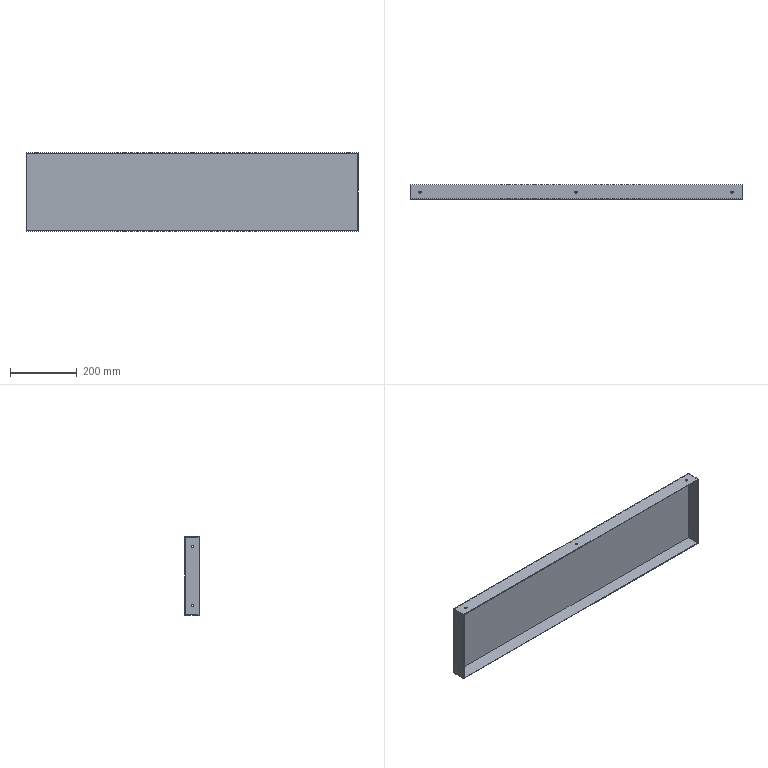Component | SolidWorks | RearCoverPlate-1 | 1 solid | 25 faces | box 993 x 42 x 235 mm | volume 662011 mm3 | cylinder 14 | plane 11 | commonest cylinder face diameters 7 x14
build123d program:
from build123d import *

# Parameters (mm, degrees)
SKETCH1_W           = 993
SKETCH1_H           = 235
BOSS_EXTRUDE1_DEPTH = 42
SHELL1_T            = -2
CUT_EXTRUDE1_REACH  = 1014.201
SKETCH2_R           = 3.5
SKETCH4_R           = 3.5
CUT_EXTRUDE3_DEPTH  = 2


with BuildPart() as part:
    # Sketch1 → Boss-Extrude1 (new body)
    with BuildSketch(Plane.XY):
        with Locations((423.284, 74.173)):
            Rectangle(SKETCH1_W, SKETCH1_H)
    extrude(amount=BOSS_EXTRUDE1_DEPTH)

    # Shell1
    shell1_openings = [part.faces().sort_by_distance(p)[0] for p in [
        (423.284, 74.173, 0),
    ]]
    offset(amount=SHELL1_T, openings=shell1_openings, kind=Kind.INTERSECTION)

    # Cut-Extrude1: up to this face of the body (flat: up to its plane)
    cut_extrude1_end = Plane(part.part.faces().sort_by_distance((919.784, 74.173, 21))[0])
    # Sketch2 → Cut-Extrude1 (cut, up to the picked face)
    with BuildSketch(Plane.ZY.offset(73.216), mode=Mode.PRIVATE) as cut_extrude1_sk1:
        with Locations((20, 161.673)):
            Circle(SKETCH2_R)
    cut_extrude1_tool1 = split(extrude(cut_extrude1_sk1.sketch, amount=-CUT_EXTRUDE1_REACH, mode=Mode.PRIVATE), bisect_by=cut_extrude1_end, keep=Keep.BOTH, mode=Mode.PRIVATE)
    # Sketch2 → Cut-Extrude1 (cut, up to the picked face)
    with BuildSketch(Plane.ZY.offset(73.216), mode=Mode.PRIVATE) as cut_extrude1_sk2:
        with Locations((20, -13.327)):
            Circle(SKETCH2_R)
    cut_extrude1_tool2 = split(extrude(cut_extrude1_sk2.sketch, amount=-CUT_EXTRUDE1_REACH, mode=Mode.PRIVATE), bisect_by=cut_extrude1_end, keep=Keep.BOTH, mode=Mode.PRIVATE)
    add(cut_extrude1_tool1.solids().sort_by(Axis((-73.216, 161.673, 20), (1, 0, 0)))[0], mode=Mode.SUBTRACT)
    add(cut_extrude1_tool2.solids().sort_by(Axis((-73.216, -13.327, 20), (1, 0, 0)))[0], mode=Mode.SUBTRACT)

    # Sketch4 → Cut-Extrude3 (cut)
    with BuildSketch(Plane.XZ.offset(-189.673)):
        with Locations(Location((-43.216, 20, 0), (0, 0, 270))):
            Circle(SKETCH4_R)
        with Locations(Location((423.284, 20, 0), (0, 0, 270))):
            Circle(SKETCH4_R)
        with Locations(Location((889.784, 20, 0), (0, 0, 270))):
            Circle(SKETCH4_R)
    extrude(amount=-CUT_EXTRUDE3_DEPTH, mode=Mode.SUBTRACT)


solid = part.part

# Placed as in the assembly
solid = solid.moved(Location((671.234, 499.566, -640.192), (-90, 0, 180)))
STEP:
#1=COLOUR_RGB('',0.7922,0.8196,0.9333);
#2=FILL_AREA_STYLE_COLOUR('',#1);
#3=FILL_AREA_STYLE('',(#2));
#4=SURFACE_STYLE_FILL_AREA(#3);
#5=SURFACE_SIDE_STYLE('',(#4));
#6=SURFACE_STYLE_USAGE(.BOTH.,#5);
#7=PRESENTATION_STYLE_ASSIGNMENT((#6));
#8=CARTESIAN_POINT('',(-8.604,20.593,-17.658));
#9=VERTEX_POINT('',#8);
#10=CARTESIAN_POINT('',(-8.604,20.318,-17.658));
#11=VERTEX_POINT('',#10);
#12=CARTESIAN_POINT('',(-8.604,20.455,-17.658));
#13=DIRECTION('',(0.,-0.,-1.));
#14=DIRECTION('',(0.,-1.,0.));
#15=AXIS2_PLACEMENT_3D('',#12,#13,#14);
#16=CIRCLE('',#15,0.1378);
#17=EDGE_CURVE('',#9,#11,#16,.T.);
#18=ORIENTED_EDGE('',*,*,#17,.F.);
#19=CARTESIAN_POINT('',(-8.604,20.593,-17.737));
#20=VERTEX_POINT('',#19);
#21=CARTESIAN_POINT('',(-8.604,20.593,-17.658));
#22=DIRECTION('',(0.,-0.,-1.));
#23=VECTOR('',#22,39.37);
#24=LINE('',#21,#23);
#25=EDGE_CURVE('',#9,#20,#24,.T.);
#26=ORIENTED_EDGE('',*,*,#25,.T.);
#27=CARTESIAN_POINT('',(-8.604,20.318,-17.737));
#28=VERTEX_POINT('',#27);
#29=CARTESIAN_POINT('',(-8.604,20.455,-17.737));
#30=DIRECTION('',(0.,-0.,-1.));
#31=DIRECTION('',(0.,-1.,0.));
#32=AXIS2_PLACEMENT_3D('',#29,#30,#31);
#33=CIRCLE('',#32,0.1378);
#34=EDGE_CURVE('',#20,#28,#33,.T.);
#35=ORIENTED_EDGE('',*,*,#34,.T.);
#36=CARTESIAN_POINT('',(-8.604,20.318,-17.658));
#37=DIRECTION('',(0.,-0.,-1.));
#38=VECTOR('',#37,39.37);
#39=LINE('',#36,#38);
#40=EDGE_CURVE('',#11,#28,#39,.T.);
#41=ORIENTED_EDGE('',*,*,#40,.F.);
#42=EDGE_LOOP('',(#18,#26,#35,#41));
#43=FACE_OUTER_BOUND('',#42,.T.);
#44=CARTESIAN_POINT('',(-8.604,20.455,-17.658));
#45=DIRECTION('',(0.,-0.,-1.));
#46=DIRECTION('',(0.,-1.,0.));
#47=AXIS2_PLACEMENT_3D('',#44,#45,#46);
#48=CYLINDRICAL_SURFACE('',#47,0.1378);
#49=ADVANCED_FACE('',(#43),#48,.F.);
#50=CARTESIAN_POINT('',(9.762,20.593,-17.658));
#51=VERTEX_POINT('',#50);
#52=CARTESIAN_POINT('',(9.762,20.318,-17.658));
#53=VERTEX_POINT('',#52);
#54=CARTESIAN_POINT('',(9.762,20.455,-17.658));
#55=DIRECTION('',(0.,-0.,-1.));
#56=DIRECTION('',(0.,-1.,0.));
#57=AXIS2_PLACEMENT_3D('',#54,#55,#56);
#58=CIRCLE('',#57,0.1378);
#59=EDGE_CURVE('',#51,#53,#58,.T.);
#60=ORIENTED_EDGE('',*,*,#59,.F.);
#61=CARTESIAN_POINT('',(9.762,20.593,-17.737));
#62=VERTEX_POINT('',#61);
#63=CARTESIAN_POINT('',(9.762,20.593,-17.658));
#64=DIRECTION('',(0.,-0.,-1.));
#65=VECTOR('',#64,39.37);
#66=LINE('',#63,#65);
#67=EDGE_CURVE('',#51,#62,#66,.T.);
#68=ORIENTED_EDGE('',*,*,#67,.T.);
#69=CARTESIAN_POINT('',(9.762,20.318,-17.737));
#70=VERTEX_POINT('',#69);
#71=CARTESIAN_POINT('',(9.762,20.455,-17.737));
#72=DIRECTION('',(0.,-0.,-1.));
#73=DIRECTION('',(0.,-1.,0.));
#74=AXIS2_PLACEMENT_3D('',#71,#72,#73);
#75=CIRCLE('',#74,0.1378);
#76=EDGE_CURVE('',#62,#70,#75,.T.);
#77=ORIENTED_EDGE('',*,*,#76,.T.);
#78=CARTESIAN_POINT('',(9.762,20.318,-17.658));
#79=DIRECTION('',(0.,-0.,-1.));
#80=VECTOR('',#79,39.37);
#81=LINE('',#78,#80);
#82=EDGE_CURVE('',#53,#70,#81,.T.);
#83=ORIENTED_EDGE('',*,*,#82,.F.);
#84=EDGE_LOOP('',(#60,#68,#77,#83));
#85=FACE_OUTER_BOUND('',#84,.T.);
#86=CARTESIAN_POINT('',(9.762,20.455,-17.658));
#87=DIRECTION('',(0.,-0.,-1.));
#88=DIRECTION('',(0.,-1.,0.));
#89=AXIS2_PLACEMENT_3D('',#86,#87,#88);
#90=CYLINDRICAL_SURFACE('',#89,0.1378);
#91=ADVANCED_FACE('',(#85),#90,.F.);
#92=CARTESIAN_POINT('',(28.128,20.593,-17.658));
#93=VERTEX_POINT('',#92);
#94=CARTESIAN_POINT('',(28.128,20.318,-17.658));
#95=VERTEX_POINT('',#94);
#96=CARTESIAN_POINT('',(28.128,20.455,-17.658));
#97=DIRECTION('',(0.,-0.,-1.));
#98=DIRECTION('',(0.,-1.,0.));
#99=AXIS2_PLACEMENT_3D('',#96,#97,#98);
#100=CIRCLE('',#99,0.1378);
#101=EDGE_CURVE('',#93,#95,#100,.T.);
#102=ORIENTED_EDGE('',*,*,#101,.F.);
#103=CARTESIAN_POINT('',(28.128,20.593,-17.737));
#104=VERTEX_POINT('',#103);
#105=CARTESIAN_POINT('',(28.128,20.593,-17.658));
#106=DIRECTION('',(0.,-0.,-1.));
#107=VECTOR('',#106,39.37);
#108=LINE('',#105,#107);
#109=EDGE_CURVE('',#93,#104,#108,.T.);
#110=ORIENTED_EDGE('',*,*,#109,.T.);
#111=CARTESIAN_POINT('',(28.128,20.318,-17.737));
#112=VERTEX_POINT('',#111);
#113=CARTESIAN_POINT('',(28.128,20.455,-17.737));
#114=DIRECTION('',(0.,-0.,-1.));
#115=DIRECTION('',(0.,-1.,0.));
#116=AXIS2_PLACEMENT_3D('',#113,#114,#115);
#117=CIRCLE('',#116,0.1378);
#118=EDGE_CURVE('',#104,#112,#117,.T.);
#119=ORIENTED_EDGE('',*,*,#118,.T.);
#120=CARTESIAN_POINT('',(28.128,20.318,-17.658));
#121=DIRECTION('',(0.,-0.,-1.));
#122=VECTOR('',#121,39.37);
#123=LINE('',#120,#122);
#124=EDGE_CURVE('',#95,#112,#123,.T.);
#125=ORIENTED_EDGE('',*,*,#124,.F.);
#126=EDGE_LOOP('',(#102,#110,#119,#125));
#127=FACE_OUTER_BOUND('',#126,.T.);
#128=CARTESIAN_POINT('',(28.128,20.455,-17.658));
#129=DIRECTION('',(0.,-0.,-1.));
#130=DIRECTION('',(0.,-1.,0.));
#131=AXIS2_PLACEMENT_3D('',#128,#129,#130);
#132=CYLINDRICAL_SURFACE('',#131,0.1378);
#133=ADVANCED_FACE('',(#127),#132,.F.);
#134=CARTESIAN_POINT('',(29.23,20.455,-25.867));
#135=VERTEX_POINT('',#134);
#136=CARTESIAN_POINT('',(29.23,20.455,-25.591));
#137=VERTEX_POINT('',#136);
#138=CARTESIAN_POINT('',(29.23,20.455,-25.729));
#139=DIRECTION('',(-1.,-0.,0.));
#140=DIRECTION('',(0.,0.,1.));
#141=AXIS2_PLACEMENT_3D('',#138,#139,#140);
#142=CIRCLE('',#141,0.1378);
#143=EDGE_CURVE('',#135,#137,#142,.T.);
#144=ORIENTED_EDGE('',*,*,#143,.T.);
#145=CARTESIAN_POINT('',(29.309,20.455,-25.591));
#146=VERTEX_POINT('',#145);
#147=CARTESIAN_POINT('',(-10.175,20.455,-25.591));
#148=DIRECTION('',(1.,0.,-0.));
#149=VECTOR('',#148,39.37);
#150=LINE('',#147,#149);
#151=EDGE_CURVE('',#137,#146,#150,.T.);
#152=ORIENTED_EDGE('',*,*,#151,.T.);
#153=CARTESIAN_POINT('',(29.309,20.455,-25.867));
#154=VERTEX_POINT('',#153);
#155=CARTESIAN_POINT('',(29.309,20.455,-25.729));
#156=DIRECTION('',(1.,0.,-0.));
#157=DIRECTION('',(0.,0.,-1.));
#158=AXIS2_PLACEMENT_3D('',#155,#156,#157);
#159=CIRCLE('',#158,0.1378);
#160=EDGE_CURVE('',#146,#154,#159,.T.);
#161=ORIENTED_EDGE('',*,*,#160,.T.);
#162=CARTESIAN_POINT('',(-10.175,20.455,-25.867));
#163=DIRECTION('',(1.,0.,-0.));
#164=VECTOR('',#163,39.37);
#165=LINE('',#162,#164);
#166=EDGE_CURVE('',#135,#154,#165,.T.);
#167=ORIENTED_EDGE('',*,*,#166,.F.);
#168=EDGE_LOOP('',(#144,#152,#161,#167));
#169=FACE_OUTER_BOUND('',#168,.T.);
#170=CARTESIAN_POINT('',(-10.175,20.455,-25.729));
#171=DIRECTION('',(1.,0.,-0.));
#172=DIRECTION('',(0.,0.,-1.));
#173=AXIS2_PLACEMENT_3D('',#170,#171,#172);
#174=CYLINDRICAL_SURFACE('',#173,0.1378);
#175=ADVANCED_FACE('',(#169),#174,.F.);
#176=CARTESIAN_POINT('',(-9.785,20.455,-25.867));
#177=VERTEX_POINT('',#176);
#178=CARTESIAN_POINT('',(-9.785,20.455,-25.591));
#179=VERTEX_POINT('',#178);
#180=CARTESIAN_POINT('',(-9.785,20.455,-25.729));
#181=DIRECTION('',(-1.,-0.,-0.));
#182=DIRECTION('',(0.,1.,0.));
#183=AXIS2_PLACEMENT_3D('',#180,#181,#182);
#184=CIRCLE('',#183,0.1378);
#185=EDGE_CURVE('',#177,#179,#184,.T.);
#186=ORIENTED_EDGE('',*,*,#185,.T.);
#187=CARTESIAN_POINT('',(-9.707,20.455,-25.591));
#188=VERTEX_POINT('',#187);
#189=CARTESIAN_POINT('',(-10.175,20.455,-25.591));
#190=DIRECTION('',(1.,0.,-0.));
#191=VECTOR('',#190,39.37);
#192=LINE('',#189,#191);
#193=EDGE_CURVE('',#179,#188,#192,.T.);
#194=ORIENTED_EDGE('',*,*,#193,.T.);
#195=CARTESIAN_POINT('',(-9.707,20.455,-25.867));
#196=VERTEX_POINT('',#195);
#197=CARTESIAN_POINT('',(-9.707,20.455,-25.729));
#198=DIRECTION('',(1.,0.,0.));
#199=DIRECTION('',(0.,1.,0.));
#200=AXIS2_PLACEMENT_3D('',#197,#198,#199);
#201=CIRCLE('',#200,0.1378);
#202=EDGE_CURVE('',#188,#196,#201,.T.);
#203=ORIENTED_EDGE('',*,*,#202,.T.);
#204=CARTESIAN_POINT('',(-10.175,20.455,-25.867));
#205=DIRECTION('',(1.,0.,-0.));
#206=VECTOR('',#205,39.37);
#207=LINE('',#204,#206);
#208=EDGE_CURVE('',#177,#196,#207,.T.);
#209=ORIENTED_EDGE('',*,*,#208,.F.);
#210=EDGE_LOOP('',(#186,#194,#203,#209));
#211=FACE_OUTER_BOUND('',#210,.T.);
#212=CARTESIAN_POINT('',(-10.175,20.455,-25.729));
#213=DIRECTION('',(1.,0.,-0.));
#214=DIRECTION('',(0.,0.,-1.));
#215=AXIS2_PLACEMENT_3D('',#212,#213,#214);
#216=CYLINDRICAL_SURFACE('',#215,0.1378);
#217=ADVANCED_FACE('',(#211),#216,.F.);
#218=CARTESIAN_POINT('',(29.23,20.455,-18.977));
#219=VERTEX_POINT('',#218);
#220=CARTESIAN_POINT('',(29.23,20.455,-18.702));
#221=VERTEX_POINT('',#220);
#222=CARTESIAN_POINT('',(29.23,20.455,-18.839));
#223=DIRECTION('',(-1.,-0.,0.));
#224=DIRECTION('',(0.,0.,1.));
#225=AXIS2_PLACEMENT_3D('',#222,#223,#224);
#226=CIRCLE('',#225,0.1378);
#227=EDGE_CURVE('',#219,#221,#226,.T.);
#228=ORIENTED_EDGE('',*,*,#227,.T.);
#229=CARTESIAN_POINT('',(29.309,20.455,-18.702));
#230=VERTEX_POINT('',#229);
#231=CARTESIAN_POINT('',(-10.175,20.455,-18.702));
#232=DIRECTION('',(1.,0.,-0.));
#233=VECTOR('',#232,39.37);
#234=LINE('',#231,#233);
#235=EDGE_CURVE('',#221,#230,#234,.T.);
#236=ORIENTED_EDGE('',*,*,#235,.T.);
#237=CARTESIAN_POINT('',(29.309,20.455,-18.977));
#238=VERTEX_POINT('',#237);
#239=CARTESIAN_POINT('',(29.309,20.455,-18.839));
#240=DIRECTION('',(1.,0.,-0.));
#241=DIRECTION('',(0.,0.,-1.));
#242=AXIS2_PLACEMENT_3D('',#239,#240,#241);
#243=CIRCLE('',#242,0.1378);
#244=EDGE_CURVE('',#230,#238,#243,.T.);
#245=ORIENTED_EDGE('',*,*,#244,.T.);
#246=CARTESIAN_POINT('',(-10.175,20.455,-18.977));
#247=DIRECTION('',(1.,0.,-0.));
#248=VECTOR('',#247,39.37);
#249=LINE('',#246,#248);
#250=EDGE_CURVE('',#219,#238,#249,.T.);
#251=ORIENTED_EDGE('',*,*,#250,.F.);
#252=EDGE_LOOP('',(#228,#236,#245,#251));
#253=FACE_OUTER_BOUND('',#252,.T.);
#254=CARTESIAN_POINT('',(-10.175,20.455,-18.839));
#255=DIRECTION('',(1.,0.,-0.));
#256=DIRECTION('',(0.,0.,-1.));
#257=AXIS2_PLACEMENT_3D('',#254,#255,#256);
#258=CYLINDRICAL_SURFACE('',#257,0.1378);
#259=ADVANCED_FACE('',(#253),#258,.F.);
#260=CARTESIAN_POINT('',(-9.785,20.455,-18.977));
#261=VERTEX_POINT('',#260);
#262=CARTESIAN_POINT('',(-9.785,20.455,-18.702));
#263=VERTEX_POINT('',#262);
#264=CARTESIAN_POINT('',(-9.785,20.455,-18.839));
#265=DIRECTION('',(-1.,-0.,-0.));
#266=DIRECTION('',(0.,1.,0.));
#267=AXIS2_PLACEMENT_3D('',#264,#265,#266);
#268=CIRCLE('',#267,0.1378);
#269=EDGE_CURVE('',#261,#263,#268,.T.);
#270=ORIENTED_EDGE('',*,*,#269,.T.);
#271=CARTESIAN_POINT('',(-9.707,20.455,-18.702));
#272=VERTEX_POINT('',#271);
#273=CARTESIAN_POINT('',(-10.175,20.455,-18.702));
#274=DIRECTION('',(1.,0.,-0.));
#275=VECTOR('',#274,39.37);
#276=LINE('',#273,#275);
#277=EDGE_CURVE('',#263,#272,#276,.T.);
#278=ORIENTED_EDGE('',*,*,#277,.T.);
#279=CARTESIAN_POINT('',(-9.707,20.455,-18.977));
#280=VERTEX_POINT('',#279);
#281=CARTESIAN_POINT('',(-9.707,20.455,-18.839));
#282=DIRECTION('',(1.,0.,0.));
#283=DIRECTION('',(0.,1.,0.));
#284=AXIS2_PLACEMENT_3D('',#281,#282,#283);
#285=CIRCLE('',#284,0.1378);
#286=EDGE_CURVE('',#272,#280,#285,.T.);
#287=ORIENTED_EDGE('',*,*,#286,.T.);
#288=CARTESIAN_POINT('',(-10.175,20.455,-18.977));
#289=DIRECTION('',(1.,0.,-0.));
#290=VECTOR('',#289,39.37);
#291=LINE('',#288,#290);
#292=EDGE_CURVE('',#261,#280,#291,.T.);
#293=ORIENTED_EDGE('',*,*,#292,.F.);
#294=EDGE_LOOP('',(#270,#278,#287,#293));
#295=FACE_OUTER_BOUND('',#294,.T.);
#296=CARTESIAN_POINT('',(-10.175,20.455,-18.839));
#297=DIRECTION('',(1.,0.,-0.));
#298=DIRECTION('',(0.,0.,-1.));
#299=AXIS2_PLACEMENT_3D('',#296,#297,#298);
#300=CYLINDRICAL_SURFACE('',#299,0.1378);
#301=ADVANCED_FACE('',(#295),#300,.F.);
#302=CARTESIAN_POINT('',(29.309,20.455,-25.729));
#303=DIRECTION('',(1.,0.,-0.));
#304=DIRECTION('',(0.,0.,-1.));
#305=AXIS2_PLACEMENT_3D('',#302,#303,#304);
#306=CIRCLE('',#305,0.1378);
#307=EDGE_CURVE('',#154,#146,#306,.T.);
#308=ORIENTED_EDGE('',*,*,#307,.F.);
#309=ORIENTED_EDGE('',*,*,#160,.F.);
#310=EDGE_LOOP('',(#308,#309));
#311=FACE_BOUND('',#310,.T.);
#312=CARTESIAN_POINT('',(29.309,20.455,-18.839));
#313=DIRECTION('',(1.,0.,-0.));
#314=DIRECTION('',(0.,0.,-1.));
#315=AXIS2_PLACEMENT_3D('',#312,#313,#314);
#316=CIRCLE('',#315,0.1378);
#317=EDGE_CURVE('',#238,#230,#316,.T.);
#318=ORIENTED_EDGE('',*,*,#317,.F.);
#319=ORIENTED_EDGE('',*,*,#244,.F.);
#320=EDGE_LOOP('',(#318,#319));
#321=FACE_BOUND('',#320,.T.);
#322=CARTESIAN_POINT('',(29.309,19.668,-17.658));
#323=VERTEX_POINT('',#322);
#324=CARTESIAN_POINT('',(29.309,19.668,-26.91));
#325=VERTEX_POINT('',#324);
#326=CARTESIAN_POINT('',(29.309,19.668,-17.658));
#327=DIRECTION('',(-0.,-0.,-1.));
#328=VECTOR('',#327,39.37);
#329=LINE('',#326,#328);
#330=EDGE_CURVE('',#323,#325,#329,.T.);
#331=ORIENTED_EDGE('',*,*,#330,.T.);
#332=CARTESIAN_POINT('',(29.309,21.322,-26.91));
#333=VERTEX_POINT('',#332);
#334=CARTESIAN_POINT('',(29.309,21.322,-26.91));
#335=DIRECTION('',(0.,-1.,0.));
#336=VECTOR('',#335,39.37);
#337=LINE('',#334,#336);
#338=EDGE_CURVE('',#333,#325,#337,.T.);
#339=ORIENTED_EDGE('',*,*,#338,.F.);
#340=CARTESIAN_POINT('',(29.309,21.322,-17.658));
#341=VERTEX_POINT('',#340);
#342=CARTESIAN_POINT('',(29.309,21.322,-17.658));
#343=DIRECTION('',(-0.,-0.,-1.));
#344=VECTOR('',#343,39.37);
#345=LINE('',#342,#344);
#346=EDGE_CURVE('',#341,#333,#345,.T.);
#347=ORIENTED_EDGE('',*,*,#346,.F.);
#348=CARTESIAN_POINT('',(29.309,21.322,-17.658));
#349=DIRECTION('',(0.,-1.,0.));
#350=VECTOR('',#349,39.37);
#351=LINE('',#348,#350);
#352=EDGE_CURVE('',#341,#323,#351,.T.);
#353=ORIENTED_EDGE('',*,*,#352,.T.);
#354=EDGE_LOOP('',(#331,#339,#347,#353));
#355=FACE_OUTER_BOUND('',#354,.T.);
#356=CARTESIAN_POINT('',(29.309,21.322,-17.658));
#357=DIRECTION('',(-1.,-0.,0.));
#358=DIRECTION('',(0.,0.,1.));
#359=AXIS2_PLACEMENT_3D('',#356,#357,#358);
#360=PLANE('',#359);
#361=ADVANCED_FACE('',(#311,#321,#355),#360,.F.);
#362=CARTESIAN_POINT('',(-9.785,19.668,-26.91));
#363=VERTEX_POINT('',#362);
#364=CARTESIAN_POINT('',(29.309,19.668,-26.91));
#365=DIRECTION('',(-1.,-0.,-0.));
#366=VECTOR('',#365,39.37);
#367=LINE('',#364,#366);
#368=EDGE_CURVE('',#325,#363,#367,.T.);
#369=ORIENTED_EDGE('',*,*,#368,.T.);
#370=CARTESIAN_POINT('',(-9.785,21.322,-26.91));
#371=VERTEX_POINT('',#370);
#372=CARTESIAN_POINT('',(-9.785,21.322,-26.91));
#373=DIRECTION('',(0.,-1.,0.));
#374=VECTOR('',#373,39.37);
#375=LINE('',#372,#374);
#376=EDGE_CURVE('',#371,#363,#375,.T.);
#377=ORIENTED_EDGE('',*,*,#376,.F.);
#378=CARTESIAN_POINT('',(29.309,21.322,-26.91));
#379=DIRECTION('',(-1.,-0.,-0.));
#380=VECTOR('',#379,39.37);
#381=LINE('',#378,#380);
#382=EDGE_CURVE('',#333,#371,#381,.T.);
#383=ORIENTED_EDGE('',*,*,#382,.F.);
#384=ORIENTED_EDGE('',*,*,#338,.T.);
#385=EDGE_LOOP('',(#369,#377,#383,#384));
#386=FACE_OUTER_BOUND('',#385,.T.);
#387=CARTESIAN_POINT('',(29.309,21.322,-26.91));
#388=DIRECTION('',(-0.,0.,1.));
#389=DIRECTION('',(0.,1.,0.));
#390=AXIS2_PLACEMENT_3D('',#387,#388,#389);
#391=PLANE('',#390);
#392=ADVANCED_FACE('',(#386),#391,.F.);
#393=ORIENTED_EDGE('',*,*,#185,.F.);
#394=CARTESIAN_POINT('',(-9.785,20.455,-25.729));
#395=DIRECTION('',(-1.,-0.,-0.));
#396=DIRECTION('',(0.,1.,0.));
#397=AXIS2_PLACEMENT_3D('',#394,#395,#396);
#398=CIRCLE('',#397,0.1378);
#399=EDGE_CURVE('',#179,#177,#398,.T.);
#400=ORIENTED_EDGE('',*,*,#399,.F.);
#401=EDGE_LOOP('',(#393,#400));
#402=FACE_BOUND('',#401,.T.);
#403=ORIENTED_EDGE('',*,*,#269,.F.);
#404=CARTESIAN_POINT('',(-9.785,20.455,-18.839));
#405=DIRECTION('',(-1.,-0.,-0.));
#406=DIRECTION('',(0.,1.,0.));
#407=AXIS2_PLACEMENT_3D('',#404,#405,#406);
#408=CIRCLE('',#407,0.1378);
#409=EDGE_CURVE('',#263,#261,#408,.T.);
#410=ORIENTED_EDGE('',*,*,#409,.F.);
#411=EDGE_LOOP('',(#403,#410));
#412=FACE_BOUND('',#411,.T.);
#413=CARTESIAN_POINT('',(-9.785,19.668,-17.658));
#414=VERTEX_POINT('',#413);
#415=CARTESIAN_POINT('',(-9.785,19.668,-17.658));
#416=DIRECTION('',(-0.,0.,1.));
#417=VECTOR('',#416,39.37);
#418=LINE('',#415,#417);
#419=EDGE_CURVE('',#363,#414,#418,.T.);
#420=ORIENTED_EDGE('',*,*,#419,.T.);
#421=CARTESIAN_POINT('',(-9.785,21.322,-17.658));
#422=VERTEX_POINT('',#421);
#423=CARTESIAN_POINT('',(-9.785,21.322,-17.658));
#424=DIRECTION('',(0.,-1.,0.));
#425=VECTOR('',#424,39.37);
#426=LINE('',#423,#425);
#427=EDGE_CURVE('',#422,#414,#426,.T.);
#428=ORIENTED_EDGE('',*,*,#427,.F.);
#429=CARTESIAN_POINT('',(-9.785,21.322,-17.658));
#430=DIRECTION('',(-0.,0.,1.));
#431=VECTOR('',#430,39.37);
#432=LINE('',#429,#431);
#433=EDGE_CURVE('',#371,#422,#432,.T.);
#434=ORIENTED_EDGE('',*,*,#433,.F.);
#435=ORIENTED_EDGE('',*,*,#376,.T.);
#436=EDGE_LOOP('',(#420,#428,#434,#435));
#437=FACE_OUTER_BOUND('',#436,.T.);
#438=CARTESIAN_POINT('',(-9.785,21.322,-17.658));
#439=DIRECTION('',(1.,0.,0.));
#440=DIRECTION('',(0.,1.,0.));
#441=AXIS2_PLACEMENT_3D('',#438,#439,#440);
#442=PLANE('',#441);
#443=ADVANCED_FACE('',(#402,#412,#437),#442,.F.);
#444=CARTESIAN_POINT('',(-8.604,20.455,-17.658));
#445=DIRECTION('',(0.,-0.,-1.));
#446=DIRECTION('',(0.,-1.,0.));
#447=AXIS2_PLACEMENT_3D('',#444,#445,#446);
#448=CIRCLE('',#447,0.1378);
#449=EDGE_CURVE('',#11,#9,#448,.T.);
#450=ORIENTED_EDGE('',*,*,#449,.T.);
#451=ORIENTED_EDGE('',*,*,#17,.T.);
#452=EDGE_LOOP('',(#450,#451));
#453=FACE_BOUND('',#452,.T.);
#454=CARTESIAN_POINT('',(9.762,20.455,-17.658));
#455=DIRECTION('',(0.,-0.,-1.));
#456=DIRECTION('',(0.,-1.,0.));
#457=AXIS2_PLACEMENT_3D('',#454,#455,#456);
#458=CIRCLE('',#457,0.1378);
#459=EDGE_CURVE('',#53,#51,#458,.T.);
#460=ORIENTED_EDGE('',*,*,#459,.T.);
#461=ORIENTED_EDGE('',*,*,#59,.T.);
#462=EDGE_LOOP('',(#460,#461));
#463=FACE_BOUND('',#462,.T.);
#464=CARTESIAN_POINT('',(28.128,20.455,-17.658));
#465=DIRECTION('',(0.,-0.,-1.));
#466=DIRECTION('',(0.,-1.,0.));
#467=AXIS2_PLACEMENT_3D('',#464,#465,#466);
#468=CIRCLE('',#467,0.1378);
#469=EDGE_CURVE('',#95,#93,#468,.T.);
#470=ORIENTED_EDGE('',*,*,#469,.T.);
#471=ORIENTED_EDGE('',*,*,#101,.T.);
#472=EDGE_LOOP('',(#470,#471));
#473=FACE_BOUND('',#472,.T.);
#474=CARTESIAN_POINT('',(29.309,19.668,-17.658));
#475=DIRECTION('',(1.,0.,0.));
#476=VECTOR('',#475,39.37);
#477=LINE('',#474,#476);
#478=EDGE_CURVE('',#414,#323,#477,.T.);
#479=ORIENTED_EDGE('',*,*,#478,.T.);
#480=ORIENTED_EDGE('',*,*,#352,.F.);
#481=CARTESIAN_POINT('',(29.309,21.322,-17.658));
#482=DIRECTION('',(1.,0.,0.));
#483=VECTOR('',#482,39.37);
#484=LINE('',#481,#483);
#485=EDGE_CURVE('',#422,#341,#484,.T.);
#486=ORIENTED_EDGE('',*,*,#485,.F.);
#487=ORIENTED_EDGE('',*,*,#427,.T.);
#488=EDGE_LOOP('',(#479,#480,#486,#487));
#489=FACE_OUTER_BOUND('',#488,.T.);
#490=CARTESIAN_POINT('',(29.309,21.322,-17.658));
#491=DIRECTION('',(0.,0.,-1.));
#492=DIRECTION('',(0.,-1.,0.));
#493=AXIS2_PLACEMENT_3D('',#490,#491,#492);
#494=PLANE('',#493);
#495=ADVANCED_FACE('',(#453,#463,#473,#489),#494,.F.);
#496=ORIENTED_EDGE('',*,*,#346,.T.);
#497=ORIENTED_EDGE('',*,*,#382,.T.);
#498=ORIENTED_EDGE('',*,*,#433,.T.);
#499=ORIENTED_EDGE('',*,*,#485,.T.);
#500=EDGE_LOOP('',(#496,#497,#498,#499));
#501=FACE_OUTER_BOUND('',#500,.T.);
#502=CARTESIAN_POINT('',(26.427,21.322,-25.204));
#503=DIRECTION('',(-0.,1.,-0.));
#504=DIRECTION('',(-1.,-0.,-0.));
#505=AXIS2_PLACEMENT_3D('',#502,#503,#504);
#506=PLANE('',#505);
#507=ADVANCED_FACE('',(#501),#506,.T.);
#508=CARTESIAN_POINT('',(-9.707,19.668,-17.737));
#509=VERTEX_POINT('',#508);
#510=CARTESIAN_POINT('',(29.23,19.668,-17.737));
#511=VERTEX_POINT('',#510);
#512=CARTESIAN_POINT('',(29.309,19.668,-17.737));
#513=DIRECTION('',(1.,0.,0.));
#514=VECTOR('',#513,39.37);
#515=LINE('',#512,#514);
#516=EDGE_CURVE('',#509,#511,#515,.T.);
#517=ORIENTED_EDGE('',*,*,#516,.T.);
#518=CARTESIAN_POINT('',(29.23,19.668,-26.831));
#519=VERTEX_POINT('',#518);
#520=CARTESIAN_POINT('',(29.23,19.668,-17.658));
#521=DIRECTION('',(-0.,-0.,-1.));
#522=VECTOR('',#521,39.37);
#523=LINE('',#520,#522);
#524=EDGE_CURVE('',#511,#519,#523,.T.);
#525=ORIENTED_EDGE('',*,*,#524,.T.);
#526=CARTESIAN_POINT('',(-9.707,19.668,-26.831));
#527=VERTEX_POINT('',#526);
#528=CARTESIAN_POINT('',(29.309,19.668,-26.831));
#529=DIRECTION('',(-1.,-0.,-0.));
#530=VECTOR('',#529,39.37);
#531=LINE('',#528,#530);
#532=EDGE_CURVE('',#519,#527,#531,.T.);
#533=ORIENTED_EDGE('',*,*,#532,.T.);
#534=CARTESIAN_POINT('',(-9.707,19.668,-17.658));
#535=DIRECTION('',(-0.,0.,1.));
#536=VECTOR('',#535,39.37);
#537=LINE('',#534,#536);
#538=EDGE_CURVE('',#527,#509,#537,.T.);
#539=ORIENTED_EDGE('',*,*,#538,.T.);
#540=EDGE_LOOP('',(#517,#525,#533,#539));
#541=FACE_BOUND('',#540,.T.);
#542=ORIENTED_EDGE('',*,*,#330,.F.);
#543=ORIENTED_EDGE('',*,*,#478,.F.);
#544=ORIENTED_EDGE('',*,*,#419,.F.);
#545=ORIENTED_EDGE('',*,*,#368,.F.);
#546=EDGE_LOOP('',(#542,#543,#544,#545));
#547=FACE_OUTER_BOUND('',#546,.T.);
#548=CARTESIAN_POINT('',(26.427,19.668,-25.204));
#549=DIRECTION('',(-0.,1.,-0.));
#550=DIRECTION('',(-1.,-0.,-0.));
#551=AXIS2_PLACEMENT_3D('',#548,#549,#550);
#552=PLANE('',#551);
#553=ADVANCED_FACE('',(#541,#547),#552,.F.);
#554=ORIENTED_EDGE('',*,*,#143,.F.);
#555=CARTESIAN_POINT('',(29.23,20.455,-25.729));
#556=DIRECTION('',(-1.,-0.,0.));
#557=DIRECTION('',(0.,0.,1.));
#558=AXIS2_PLACEMENT_3D('',#555,#556,#557);
#559=CIRCLE('',#558,0.1378);
#560=EDGE_CURVE('',#137,#135,#559,.T.);
#561=ORIENTED_EDGE('',*,*,#560,.F.);
#562=EDGE_LOOP('',(#554,#561));
#563=FACE_BOUND('',#562,.T.);
#564=ORIENTED_EDGE('',*,*,#227,.F.);
#565=CARTESIAN_POINT('',(29.23,20.455,-18.839));
#566=DIRECTION('',(-1.,-0.,0.));
#567=DIRECTION('',(0.,0.,1.));
#568=AXIS2_PLACEMENT_3D('',#565,#566,#567);
#569=CIRCLE('',#568,0.1378);
#570=EDGE_CURVE('',#221,#219,#569,.T.);
#571=ORIENTED_EDGE('',*,*,#570,.F.);
#572=EDGE_LOOP('',(#564,#571));
#573=FACE_BOUND('',#572,.T.);
#574=ORIENTED_EDGE('',*,*,#524,.F.);
#575=CARTESIAN_POINT('',(29.23,21.243,-17.737));
#576=VERTEX_POINT('',#575);
#577=CARTESIAN_POINT('',(29.23,21.322,-17.737));
#578=DIRECTION('',(0.,-1.,0.));
#579=VECTOR('',#578,39.37);
#580=LINE('',#577,#579);
#581=EDGE_CURVE('',#576,#511,#580,.T.);
#582=ORIENTED_EDGE('',*,*,#581,.F.);
#583=CARTESIAN_POINT('',(29.23,21.243,-26.831));
#584=VERTEX_POINT('',#583);
#585=CARTESIAN_POINT('',(29.23,21.243,-17.658));
#586=DIRECTION('',(-0.,-0.,-1.));
#587=VECTOR('',#586,39.37);
#588=LINE('',#585,#587);
#589=EDGE_CURVE('',#576,#584,#588,.T.);
#590=ORIENTED_EDGE('',*,*,#589,.T.);
#591=CARTESIAN_POINT('',(29.23,21.322,-26.831));
#592=DIRECTION('',(0.,-1.,0.));
#593=VECTOR('',#592,39.37);
#594=LINE('',#591,#593);
#595=EDGE_CURVE('',#584,#519,#594,.T.);
#596=ORIENTED_EDGE('',*,*,#595,.T.);
#597=EDGE_LOOP('',(#574,#582,#590,#596));
#598=FACE_OUTER_BOUND('',#597,.T.);
#599=CARTESIAN_POINT('',(29.23,21.322,-17.658));
#600=DIRECTION('',(-1.,-0.,0.));
#601=DIRECTION('',(0.,0.,1.));
#602=AXIS2_PLACEMENT_3D('',#599,#600,#601);
#603=PLANE('',#602);
#604=ADVANCED_FACE('',(#563,#573,#598),#603,.T.);
#605=ORIENTED_EDGE('',*,*,#532,.F.);
#606=ORIENTED_EDGE('',*,*,#595,.F.);
#607=CARTESIAN_POINT('',(-9.707,21.243,-26.831));
#608=VERTEX_POINT('',#607);
#609=CARTESIAN_POINT('',(29.309,21.243,-26.831));
#610=DIRECTION('',(-1.,-0.,-0.));
#611=VECTOR('',#610,39.37);
#612=LINE('',#609,#611);
#613=EDGE_CURVE('',#584,#608,#612,.T.);
#614=ORIENTED_EDGE('',*,*,#613,.T.);
#615=CARTESIAN_POINT('',(-9.707,21.322,-26.831));
#616=DIRECTION('',(0.,-1.,0.));
#617=VECTOR('',#616,39.37);
#618=LINE('',#615,#617);
#619=EDGE_CURVE('',#608,#527,#618,.T.);
#620=ORIENTED_EDGE('',*,*,#619,.T.);
#621=EDGE_LOOP('',(#605,#606,#614,#620));
#622=FACE_OUTER_BOUND('',#621,.T.);
#623=CARTESIAN_POINT('',(29.309,21.322,-26.831));
#624=DIRECTION('',(-0.,0.,1.));
#625=DIRECTION('',(0.,1.,0.));
#626=AXIS2_PLACEMENT_3D('',#623,#624,#625);
#627=PLANE('',#626);
#628=ADVANCED_FACE('',(#622),#627,.T.);
#629=CARTESIAN_POINT('',(-9.707,20.455,-25.729));
#630=DIRECTION('',(1.,0.,0.));
#631=DIRECTION('',(0.,1.,0.));
#632=AXIS2_PLACEMENT_3D('',#629,#630,#631);
#633=CIRCLE('',#632,0.1378);
#634=EDGE_CURVE('',#196,#188,#633,.T.);
#635=ORIENTED_EDGE('',*,*,#634,.F.);
#636=ORIENTED_EDGE('',*,*,#202,.F.);
#637=EDGE_LOOP('',(#635,#636));
#638=FACE_BOUND('',#637,.T.);
#639=CARTESIAN_POINT('',(-9.707,20.455,-18.839));
#640=DIRECTION('',(1.,0.,0.));
#641=DIRECTION('',(0.,1.,0.));
#642=AXIS2_PLACEMENT_3D('',#639,#640,#641);
#643=CIRCLE('',#642,0.1378);
#644=EDGE_CURVE('',#280,#272,#643,.T.);
#645=ORIENTED_EDGE('',*,*,#644,.F.);
#646=ORIENTED_EDGE('',*,*,#286,.F.);
#647=EDGE_LOOP('',(#645,#646));
#648=FACE_BOUND('',#647,.T.);
#649=ORIENTED_EDGE('',*,*,#538,.F.);
#650=ORIENTED_EDGE('',*,*,#619,.F.);
#651=CARTESIAN_POINT('',(-9.707,21.243,-17.737));
#652=VERTEX_POINT('',#651);
#653=CARTESIAN_POINT('',(-9.707,21.243,-17.658));
#654=DIRECTION('',(-0.,0.,1.));
#655=VECTOR('',#654,39.37);
#656=LINE('',#653,#655);
#657=EDGE_CURVE('',#608,#652,#656,.T.);
#658=ORIENTED_EDGE('',*,*,#657,.T.);
#659=CARTESIAN_POINT('',(-9.707,21.322,-17.737));
#660=DIRECTION('',(0.,-1.,0.));
#661=VECTOR('',#660,39.37);
#662=LINE('',#659,#661);
#663=EDGE_CURVE('',#652,#509,#662,.T.);
#664=ORIENTED_EDGE('',*,*,#663,.T.);
#665=EDGE_LOOP('',(#649,#650,#658,#664));
#666=FACE_OUTER_BOUND('',#665,.T.);
#667=CARTESIAN_POINT('',(-9.707,21.322,-17.658));
#668=DIRECTION('',(1.,0.,0.));
#669=DIRECTION('',(0.,1.,0.));
#670=AXIS2_PLACEMENT_3D('',#667,#668,#669);
#671=PLANE('',#670);
#672=ADVANCED_FACE('',(#638,#648,#666),#671,.T.);
#673=CARTESIAN_POINT('',(-8.604,20.455,-17.737));
#674=DIRECTION('',(0.,-0.,-1.));
#675=DIRECTION('',(0.,-1.,0.));
#676=AXIS2_PLACEMENT_3D('',#673,#674,#675);
#677=CIRCLE('',#676,0.1378);
#678=EDGE_CURVE('',#28,#20,#677,.T.);
#679=ORIENTED_EDGE('',*,*,#678,.F.);
#680=ORIENTED_EDGE('',*,*,#34,.F.);
#681=EDGE_LOOP('',(#679,#680));
#682=FACE_BOUND('',#681,.T.);
#683=CARTESIAN_POINT('',(9.762,20.455,-17.737));
#684=DIRECTION('',(0.,-0.,-1.));
#685=DIRECTION('',(0.,-1.,0.));
#686=AXIS2_PLACEMENT_3D('',#683,#684,#685);
#687=CIRCLE('',#686,0.1378);
#688=EDGE_CURVE('',#70,#62,#687,.T.);
#689=ORIENTED_EDGE('',*,*,#688,.F.);
#690=ORIENTED_EDGE('',*,*,#76,.F.);
#691=EDGE_LOOP('',(#689,#690));
#692=FACE_BOUND('',#691,.T.);
#693=CARTESIAN_POINT('',(28.128,20.455,-17.737));
#694=DIRECTION('',(0.,-0.,-1.));
#695=DIRECTION('',(0.,-1.,0.));
#696=AXIS2_PLACEMENT_3D('',#693,#694,#695);
#697=CIRCLE('',#696,0.1378);
#698=EDGE_CURVE('',#112,#104,#697,.T.);
#699=ORIENTED_EDGE('',*,*,#698,.F.);
#700=ORIENTED_EDGE('',*,*,#118,.F.);
#701=EDGE_LOOP('',(#699,#700));
#702=FACE_BOUND('',#701,.T.);
#703=ORIENTED_EDGE('',*,*,#516,.F.);
#704=ORIENTED_EDGE('',*,*,#663,.F.);
#705=CARTESIAN_POINT('',(29.309,21.243,-17.737));
#706=DIRECTION('',(1.,0.,0.));
#707=VECTOR('',#706,39.37);
#708=LINE('',#705,#707);
#709=EDGE_CURVE('',#652,#576,#708,.T.);
#710=ORIENTED_EDGE('',*,*,#709,.T.);
#711=ORIENTED_EDGE('',*,*,#581,.T.);
#712=EDGE_LOOP('',(#703,#704,#710,#711));
#713=FACE_OUTER_BOUND('',#712,.T.);
#714=CARTESIAN_POINT('',(29.309,21.322,-17.737));
#715=DIRECTION('',(0.,0.,-1.));
#716=DIRECTION('',(0.,-1.,0.));
#717=AXIS2_PLACEMENT_3D('',#714,#715,#716);
#718=PLANE('',#717);
#719=ADVANCED_FACE('',(#682,#692,#702,#713),#718,.T.);
#720=ORIENTED_EDGE('',*,*,#589,.F.);
#721=ORIENTED_EDGE('',*,*,#709,.F.);
#722=ORIENTED_EDGE('',*,*,#657,.F.);
#723=ORIENTED_EDGE('',*,*,#613,.F.);
#724=EDGE_LOOP('',(#720,#721,#722,#723));
#725=FACE_OUTER_BOUND('',#724,.T.);
#726=CARTESIAN_POINT('',(26.427,21.243,-25.204));
#727=DIRECTION('',(-0.,1.,-0.));
#728=DIRECTION('',(-1.,-0.,-0.));
#729=AXIS2_PLACEMENT_3D('',#726,#727,#728);
#730=PLANE('',#729);
#731=ADVANCED_FACE('',(#725),#730,.F.);
#732=ORIENTED_EDGE('',*,*,#277,.F.);
#733=ORIENTED_EDGE('',*,*,#409,.T.);
#734=ORIENTED_EDGE('',*,*,#292,.T.);
#735=ORIENTED_EDGE('',*,*,#644,.T.);
#736=EDGE_LOOP('',(#732,#733,#734,#735));
#737=FACE_OUTER_BOUND('',#736,.T.);
#738=CARTESIAN_POINT('',(-10.175,20.455,-18.839));
#739=DIRECTION('',(1.,0.,-0.));
#740=DIRECTION('',(0.,0.,-1.));
#741=AXIS2_PLACEMENT_3D('',#738,#739,#740);
#742=CYLINDRICAL_SURFACE('',#741,0.1378);
#743=ADVANCED_FACE('',(#737),#742,.F.);
#744=ORIENTED_EDGE('',*,*,#235,.F.);
#745=ORIENTED_EDGE('',*,*,#570,.T.);
#746=ORIENTED_EDGE('',*,*,#250,.T.);
#747=ORIENTED_EDGE('',*,*,#317,.T.);
#748=EDGE_LOOP('',(#744,#745,#746,#747));
#749=FACE_OUTER_BOUND('',#748,.T.);
#750=CARTESIAN_POINT('',(-10.175,20.455,-18.839));
#751=DIRECTION('',(1.,0.,-0.));
#752=DIRECTION('',(0.,0.,-1.));
#753=AXIS2_PLACEMENT_3D('',#750,#751,#752);
#754=CYLINDRICAL_SURFACE('',#753,0.1378);
#755=ADVANCED_FACE('',(#749),#754,.F.);
#756=ORIENTED_EDGE('',*,*,#193,.F.);
#757=ORIENTED_EDGE('',*,*,#399,.T.);
#758=ORIENTED_EDGE('',*,*,#208,.T.);
#759=ORIENTED_EDGE('',*,*,#634,.T.);
#760=EDGE_LOOP('',(#756,#757,#758,#759));
#761=FACE_OUTER_BOUND('',#760,.T.);
#762=CARTESIAN_POINT('',(-10.175,20.455,-25.729));
#763=DIRECTION('',(1.,0.,-0.));
#764=DIRECTION('',(0.,0.,-1.));
#765=AXIS2_PLACEMENT_3D('',#762,#763,#764);
#766=CYLINDRICAL_SURFACE('',#765,0.1378);
#767=ADVANCED_FACE('',(#761),#766,.F.);
#768=ORIENTED_EDGE('',*,*,#151,.F.);
#769=ORIENTED_EDGE('',*,*,#560,.T.);
#770=ORIENTED_EDGE('',*,*,#166,.T.);
#771=ORIENTED_EDGE('',*,*,#307,.T.);
#772=EDGE_LOOP('',(#768,#769,#770,#771));
#773=FACE_OUTER_BOUND('',#772,.T.);
#774=CARTESIAN_POINT('',(-10.175,20.455,-25.729));
#775=DIRECTION('',(1.,0.,-0.));
#776=DIRECTION('',(0.,0.,-1.));
#777=AXIS2_PLACEMENT_3D('',#774,#775,#776);
#778=CYLINDRICAL_SURFACE('',#777,0.1378);
#779=ADVANCED_FACE('',(#773),#778,.F.);
#780=ORIENTED_EDGE('',*,*,#109,.F.);
#781=ORIENTED_EDGE('',*,*,#469,.F.);
#782=ORIENTED_EDGE('',*,*,#124,.T.);
#783=ORIENTED_EDGE('',*,*,#698,.T.);
#784=EDGE_LOOP('',(#780,#781,#782,#783));
#785=FACE_OUTER_BOUND('',#784,.T.);
#786=CARTESIAN_POINT('',(28.128,20.455,-17.658));
#787=DIRECTION('',(0.,-0.,-1.));
#788=DIRECTION('',(0.,-1.,0.));
#789=AXIS2_PLACEMENT_3D('',#786,#787,#788);
#790=CYLINDRICAL_SURFACE('',#789,0.1378);
#791=ADVANCED_FACE('',(#785),#790,.F.);
#792=ORIENTED_EDGE('',*,*,#67,.F.);
#793=ORIENTED_EDGE('',*,*,#459,.F.);
#794=ORIENTED_EDGE('',*,*,#82,.T.);
#795=ORIENTED_EDGE('',*,*,#688,.T.);
#796=EDGE_LOOP('',(#792,#793,#794,#795));
#797=FACE_OUTER_BOUND('',#796,.T.);
#798=CARTESIAN_POINT('',(9.762,20.455,-17.658));
#799=DIRECTION('',(0.,-0.,-1.));
#800=DIRECTION('',(0.,-1.,0.));
#801=AXIS2_PLACEMENT_3D('',#798,#799,#800);
#802=CYLINDRICAL_SURFACE('',#801,0.1378);
#803=ADVANCED_FACE('',(#797),#802,.F.);
#804=ORIENTED_EDGE('',*,*,#25,.F.);
#805=ORIENTED_EDGE('',*,*,#449,.F.);
#806=ORIENTED_EDGE('',*,*,#40,.T.);
#807=ORIENTED_EDGE('',*,*,#678,.T.);
#808=EDGE_LOOP('',(#804,#805,#806,#807));
#809=FACE_OUTER_BOUND('',#808,.T.);
#810=CARTESIAN_POINT('',(-8.604,20.455,-17.658));
#811=DIRECTION('',(0.,-0.,-1.));
#812=DIRECTION('',(0.,-1.,0.));
#813=AXIS2_PLACEMENT_3D('',#810,#811,#812);
#814=CYLINDRICAL_SURFACE('',#813,0.1378);
#815=ADVANCED_FACE('',(#809),#814,.F.);
#816=CLOSED_SHELL('',(#49,#91,#133,#175,#217,#259,#301,#361,#392,#443,#495,#507,#553,#604,#628,#672,#719,#731,#743,#755,#767,#779,#791,#803,#815));
#817=MANIFOLD_SOLID_BREP('',#816);
#818=STYLED_ITEM('',(#7),#817);
#819=(LENGTH_UNIT()NAMED_UNIT(*)SI_UNIT($,.METRE.));
#820=LENGTH_MEASURE_WITH_UNIT(LENGTH_MEASURE(0.0254),#819);
#821=DIMENSIONAL_EXPONENTS(1.,0.,0.,0.,0.,0.,0.);
#822=(CONVERSION_BASED_UNIT('',#820)LENGTH_UNIT()NAMED_UNIT(#821));
#823=UNCERTAINTY_MEASURE_WITH_UNIT(LENGTH_MEASURE(0.00001),#822,'','');
#824=(NAMED_UNIT(*)PLANE_ANGLE_UNIT()SI_UNIT($,.RADIAN.));
#825=(NAMED_UNIT(*)SI_UNIT($,.STERADIAN.)SOLID_ANGLE_UNIT());
#826=(GEOMETRIC_REPRESENTATION_CONTEXT(3)GLOBAL_UNCERTAINTY_ASSIGNED_CONTEXT((#823))GLOBAL_UNIT_ASSIGNED_CONTEXT((#822,#824,#825))REPRESENTATION_CONTEXT('',''));
#827=MECHANICAL_DESIGN_GEOMETRIC_PRESENTATION_REPRESENTATION('',(#818),#826);
#828=PRESENTATION_LAYER_ASSIGNMENT('','',(#818));
#829=CARTESIAN_POINT('',(0.,0.,0.));
#830=DIRECTION('',(0.,0.,1.));
#831=DIRECTION('',(1.,0.,0.));
#832=AXIS2_PLACEMENT_3D('',#829,#830,#831);
#833=(LENGTH_UNIT()NAMED_UNIT(*)SI_UNIT($,.METRE.));
#834=LENGTH_MEASURE_WITH_UNIT(LENGTH_MEASURE(0.0254),#833);
#835=DIMENSIONAL_EXPONENTS(1.,0.,0.,0.,0.,0.,0.);
#836=(CONVERSION_BASED_UNIT('',#834)LENGTH_UNIT()NAMED_UNIT(#835));
#837=UNCERTAINTY_MEASURE_WITH_UNIT(LENGTH_MEASURE(0.00001),#836,'','');
#838=(NAMED_UNIT(*)PLANE_ANGLE_UNIT()SI_UNIT($,.RADIAN.));
#839=(NAMED_UNIT(*)SI_UNIT($,.STERADIAN.)SOLID_ANGLE_UNIT());
#840=(GEOMETRIC_REPRESENTATION_CONTEXT(3)GLOBAL_UNCERTAINTY_ASSIGNED_CONTEXT((#837))GLOBAL_UNIT_ASSIGNED_CONTEXT((#836,#838,#839))REPRESENTATION_CONTEXT('',''));
#841=ADVANCED_BREP_SHAPE_REPRESENTATION('',(#817,#832),#840);